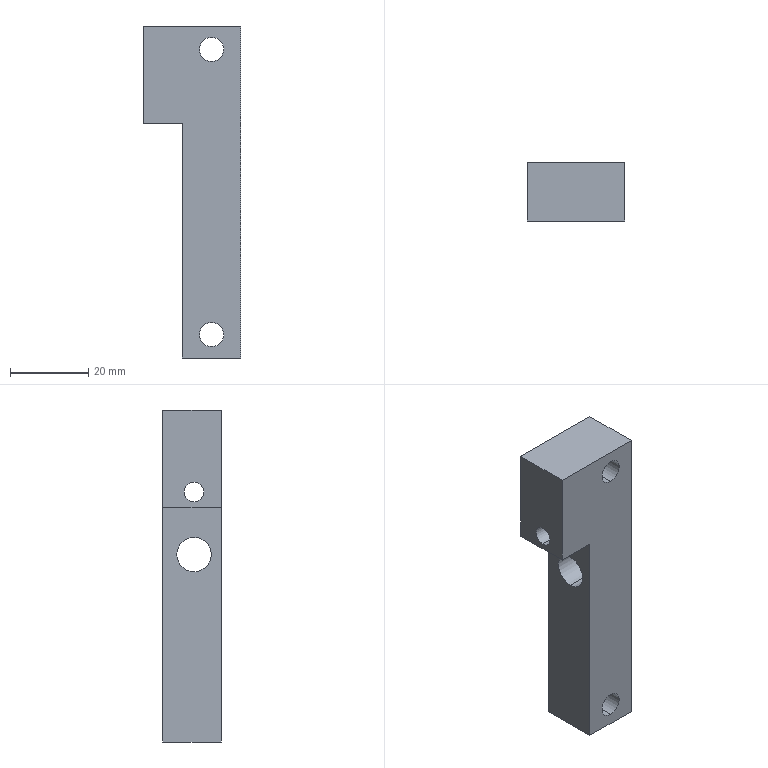CAM job | Mastercam | mm | 12 operations | part box 25 x 15 x 85
1. Facing | 20 - 63 平铣刀
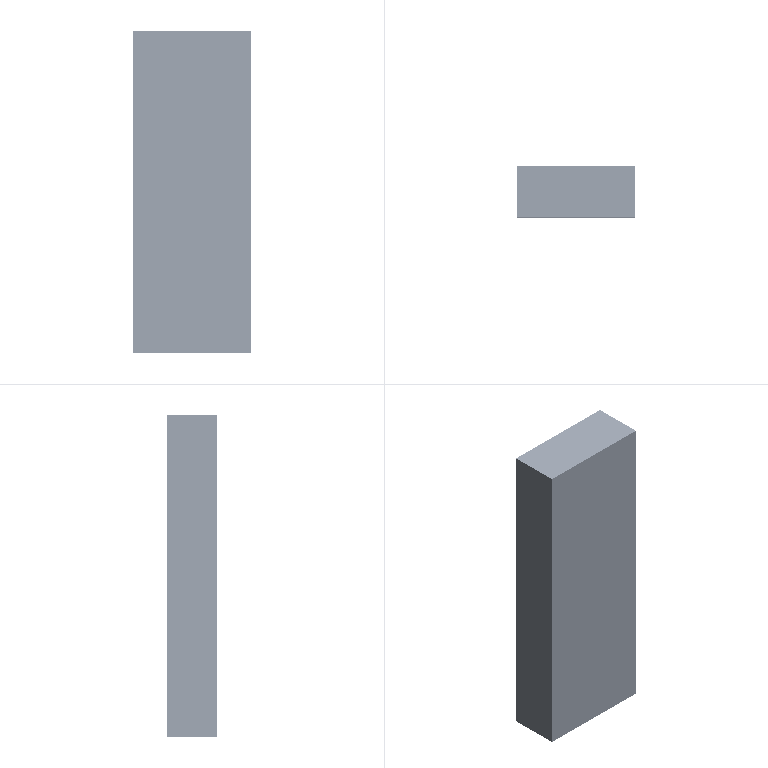2. Contour (Ramp) | 10 - 10 平铣刀
3. Contour (2D) | 10 - 10 平铣刀
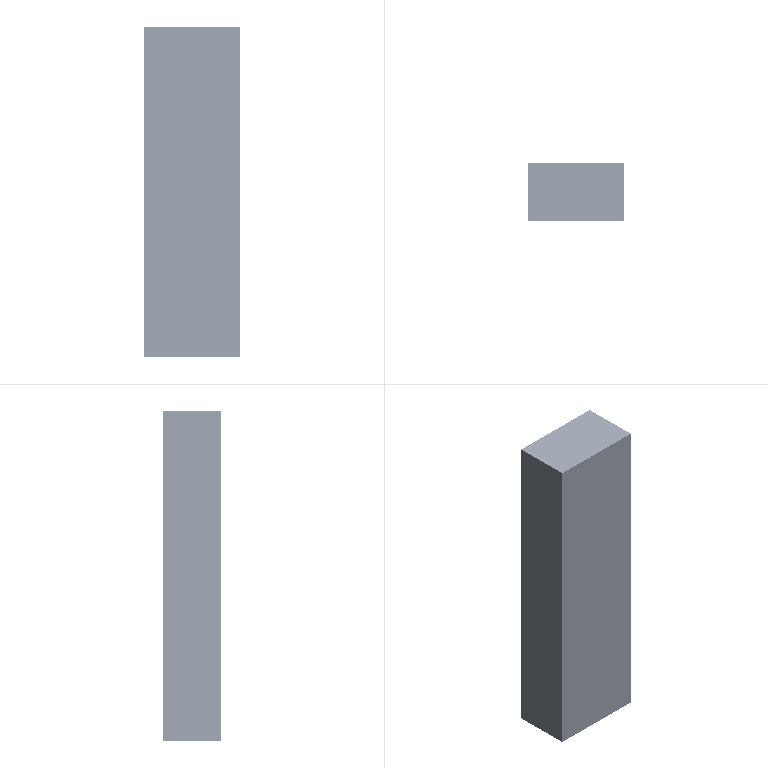4. Drill/Counterbore | 7 - 4 倒角刀
5. Contour (2D chamfer) | 7 - 4 倒角刀
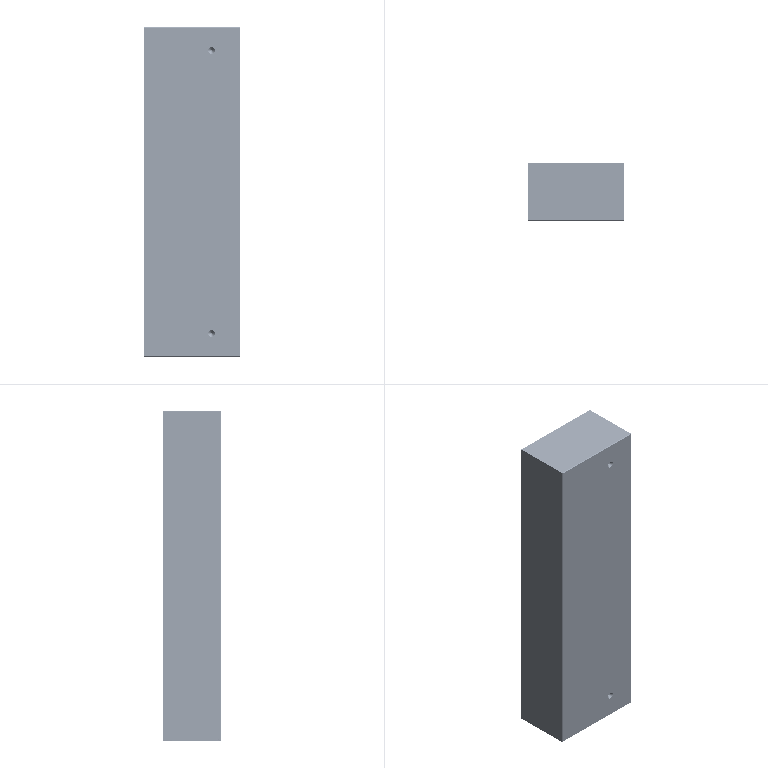6. Facing | 20 - 63 平铣刀
7. Contour (2D chamfer) | 7 - 4 倒角刀
8. Contour (2D) | 10 - 10 平铣刀
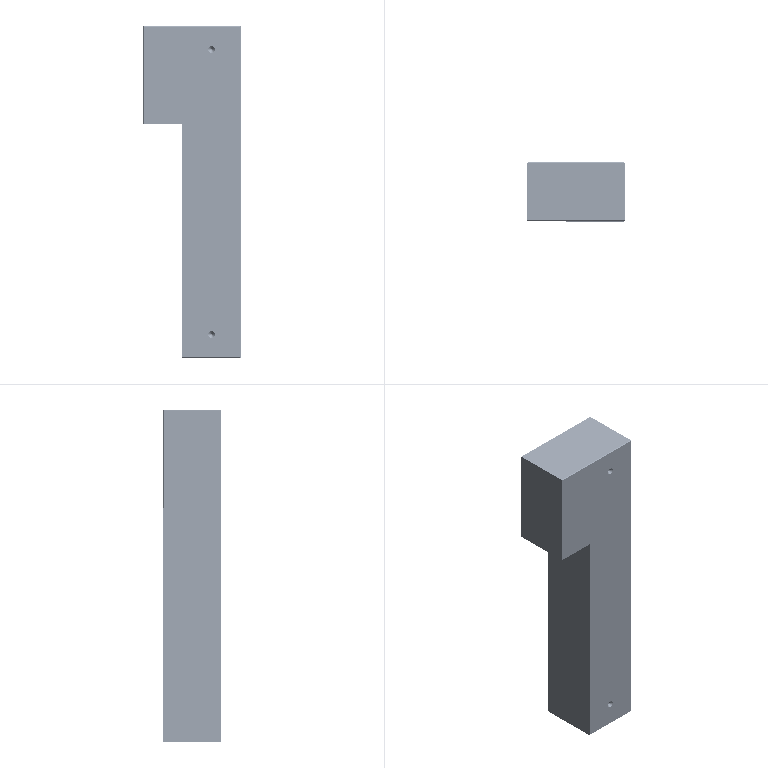9. Contour (2D) | 10 - 10 平铣刀
10. Drill/Counterbore | 7 - 4 倒角刀
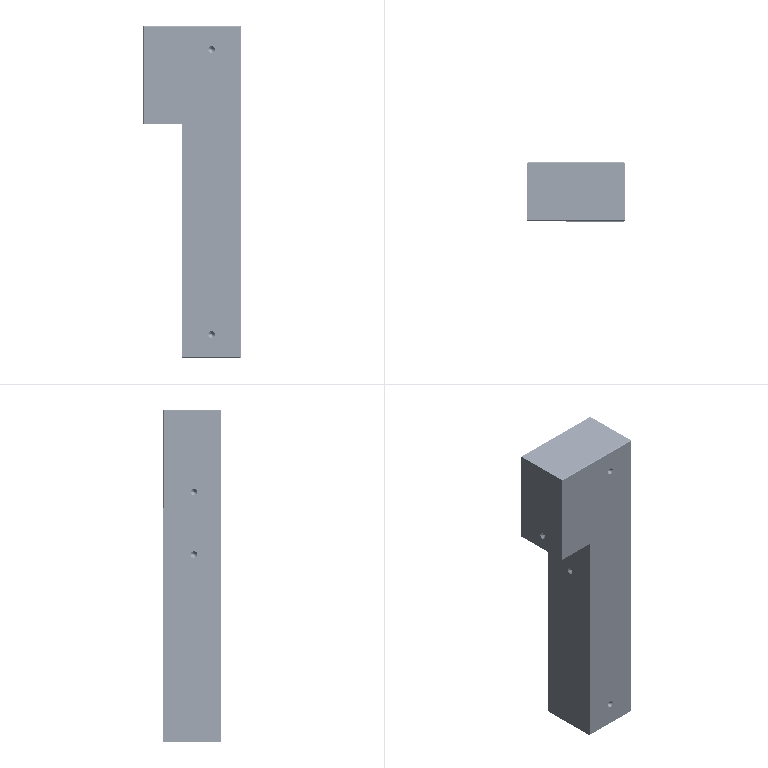11. Contour (2D chamfer) | 7 - 4 倒角刀
12. Contour (2D chamfer) | 7 - 4 倒角刀